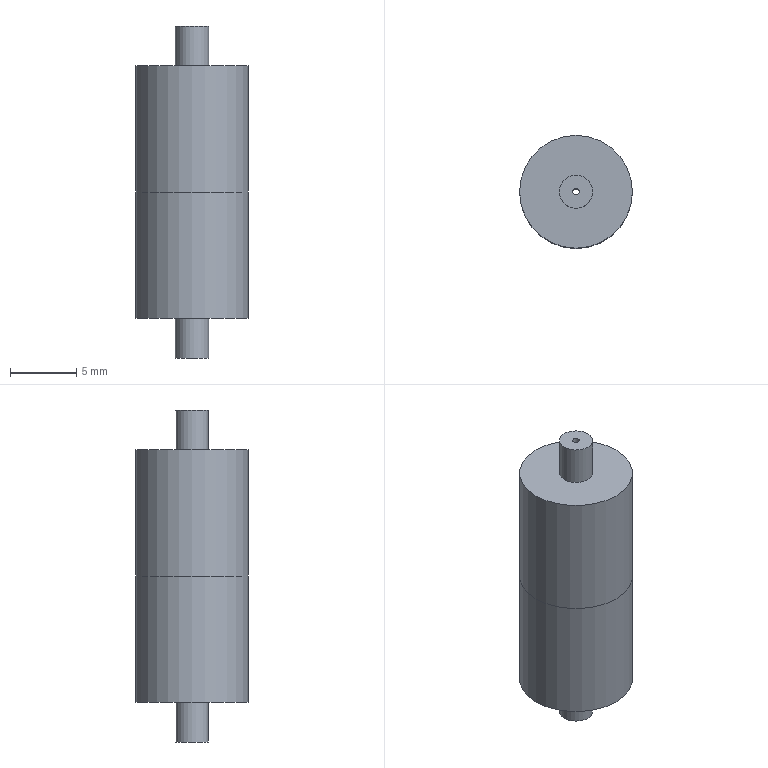Component | NX | MODEL6 | 2 solids | 12 faces | box 8.49 x 8.49 x 25 mm | volume 1101 mm3 | plane 6 | cylinder 6 | commonest cylinder face diameters 8.493 x2 0.493 x2 2.493 x2
STEP:
#1=CARTESIAN_POINT('',(0.,0.,0.));
#2=DIRECTION('',(0.,0.,1.));
#3=DIRECTION('',(1.,0.,0.));
#4=AXIS2_PLACEMENT_3D('',#1,#2,#3);
#5=CARTESIAN_POINT('',(86.254,-6.878,25.));
#6=VERTEX_POINT('',#5);
#7=CARTESIAN_POINT('',(90.5,-6.878,25.));
#8=DIRECTION('',(0.,0.,-1.));
#9=DIRECTION('',(-1.,0.,0.));
#10=AXIS2_PLACEMENT_3D('',#7,#8,#9);
#11=CIRCLE('',#10,4.247);
#12=CARTESIAN_POINT('',(90.5,-5.631,25.));
#13=DIRECTION('',(0.,0.,1.));
#14=DIRECTION('',(-1.,0.,0.));
#15=AXIS2_PLACEMENT_3D('',#12,#13,#14);
#16=PLANE('',#15);
#17=CARTESIAN_POINT('',(4.247,1.247));
#18=CARTESIAN_POINT('',(4.247,-6.109));
#19=CARTESIAN_POINT('',(-2.123,-2.431));
#20=CARTESIAN_POINT('',(-8.493,1.247));
#21=CARTESIAN_POINT('',(-2.123,4.925));
#22=CARTESIAN_POINT('',(4.247,8.602));
#23=CARTESIAN_POINT('',(4.247,1.247));
#24=(BOUNDED_CURVE()B_SPLINE_CURVE(2,(#17,#18,#19,#20,#21,#22,#23),.UNSPECIFIED.,.T.,.F.)B_SPLINE_CURVE_WITH_KNOTS((1,2,2,2,2,1),(-2.094,0.,2.094,4.189,6.283,8.378),.UNSPECIFIED.)CURVE()GEOMETRIC_REPRESENTATION_ITEM()RATIONAL_B_SPLINE_CURVE((1.,0.5,1.,0.5,1.,0.5,1.))REPRESENTATION_ITEM(''));
#25=(GEOMETRIC_REPRESENTATION_CONTEXT(2)PARAMETRIC_REPRESENTATION_CONTEXT()REPRESENTATION_CONTEXT('',''));
#26=DEFINITIONAL_REPRESENTATION('',(#24),#25);
#27=PCURVE('',#16,#26);
#28=CARTESIAN_POINT('',(90.5,-6.878,26.72));
#29=DIRECTION('',(0.,0.,1.));
#30=DIRECTION('',(-1.,0.,0.));
#31=AXIS2_PLACEMENT_3D('',#28,#29,#30);
#32=CYLINDRICAL_SURFACE('',#31,4.247);
#33=CARTESIAN_POINT('',(6.283,-1.72));
#34=DIRECTION('',(-1.,0.));
#35=VECTOR('',#34,1.);
#36=LINE('',#33,#35);
#37=(GEOMETRIC_REPRESENTATION_CONTEXT(2)PARAMETRIC_REPRESENTATION_CONTEXT()REPRESENTATION_CONTEXT('',''));
#38=DEFINITIONAL_REPRESENTATION('',(#36),#37);
#39=PCURVE('',#32,#38);
#40=SURFACE_CURVE('',#11,(#27,#39),.PCURVE_S1.);
#41=EDGE_CURVE('',#6,#6,#40,.T.);
#42=ORIENTED_EDGE('',*,*,#41,.F.);
#43=EDGE_LOOP('',(#42));
#44=FACE_BOUND('',#43,.T.);
#45=CARTESIAN_POINT('',(89.254,-6.878,25.));
#46=VERTEX_POINT('',#45);
#47=CARTESIAN_POINT('',(90.5,-6.878,25.));
#48=DIRECTION('',(0.,0.,-1.));
#49=DIRECTION('',(-1.,0.,0.));
#50=AXIS2_PLACEMENT_3D('',#47,#48,#49);
#51=CIRCLE('',#50,1.247);
#52=CARTESIAN_POINT('',(1.247,1.247));
#53=CARTESIAN_POINT('',(1.247,-0.9127));
#54=CARTESIAN_POINT('',(-0.6234,0.167));
#55=CARTESIAN_POINT('',(-2.493,1.247));
#56=CARTESIAN_POINT('',(-0.6234,2.326));
#57=CARTESIAN_POINT('',(1.247,3.406));
#58=CARTESIAN_POINT('',(1.247,1.247));
#59=(BOUNDED_CURVE()B_SPLINE_CURVE(2,(#52,#53,#54,#55,#56,#57,#58),.UNSPECIFIED.,.T.,.F.)B_SPLINE_CURVE_WITH_KNOTS((1,2,2,2,2,1),(-2.094,0.,2.094,4.189,6.283,8.378),.UNSPECIFIED.)CURVE()GEOMETRIC_REPRESENTATION_ITEM()RATIONAL_B_SPLINE_CURVE((1.,0.5,1.,0.5,1.,0.5,1.))REPRESENTATION_ITEM(''));
#60=(GEOMETRIC_REPRESENTATION_CONTEXT(2)PARAMETRIC_REPRESENTATION_CONTEXT()REPRESENTATION_CONTEXT('',''));
#61=DEFINITIONAL_REPRESENTATION('',(#59),#60);
#62=PCURVE('',#16,#61);
#63=CARTESIAN_POINT('',(90.5,-6.878,26.72));
#64=DIRECTION('',(0.,0.,1.));
#65=DIRECTION('',(-1.,0.,0.));
#66=AXIS2_PLACEMENT_3D('',#63,#64,#65);
#67=CYLINDRICAL_SURFACE('',#66,1.247);
#68=CARTESIAN_POINT('',(6.283,-1.72));
#69=DIRECTION('',(-1.,0.));
#70=VECTOR('',#69,1.);
#71=LINE('',#68,#70);
#72=(GEOMETRIC_REPRESENTATION_CONTEXT(2)PARAMETRIC_REPRESENTATION_CONTEXT()REPRESENTATION_CONTEXT('',''));
#73=DEFINITIONAL_REPRESENTATION('',(#71),#72);
#74=PCURVE('',#67,#73);
#75=SURFACE_CURVE('',#51,(#62,#74),.PCURVE_S1.);
#76=EDGE_CURVE('',#46,#46,#75,.T.);
#77=ORIENTED_EDGE('',*,*,#76,.T.);
#78=EDGE_LOOP('',(#77));
#79=FACE_BOUND('',#78,.T.);
#80=ADVANCED_FACE('',(#44,#79),#16,.T.);
#81=CARTESIAN_POINT('',(86.254,-6.878,15.5));
#82=VERTEX_POINT('',#81);
#83=CARTESIAN_POINT('',(90.5,-6.878,15.5));
#84=DIRECTION('',(0.,0.,-1.));
#85=DIRECTION('',(-1.,0.,0.));
#86=AXIS2_PLACEMENT_3D('',#83,#84,#85);
#87=CIRCLE('',#86,4.247);
#88=CARTESIAN_POINT('',(6.283,-11.22));
#89=DIRECTION('',(-1.,0.));
#90=VECTOR('',#89,1.);
#91=LINE('',#88,#90);
#92=(GEOMETRIC_REPRESENTATION_CONTEXT(2)PARAMETRIC_REPRESENTATION_CONTEXT()REPRESENTATION_CONTEXT('',''));
#93=DEFINITIONAL_REPRESENTATION('',(#91),#92);
#94=PCURVE('',#32,#93);
#95=CARTESIAN_POINT('',(90.5,-2.631,15.5));
#96=DIRECTION('',(0.,0.,-1.));
#97=DIRECTION('',(1.,0.,0.));
#98=AXIS2_PLACEMENT_3D('',#95,#96,#97);
#99=PLANE('',#98);
#100=CARTESIAN_POINT('',(0.,4.247));
#101=DIRECTION('',(-1.,0.));
#102=AXIS2_PLACEMENT_2D('',#100,#101);
#103=CIRCLE('',#102,4.247);
#104=(GEOMETRIC_REPRESENTATION_CONTEXT(2)PARAMETRIC_REPRESENTATION_CONTEXT()REPRESENTATION_CONTEXT('',''));
#105=DEFINITIONAL_REPRESENTATION('',(#103),#104);
#106=PCURVE('',#99,#105);
#107=SURFACE_CURVE('',#87,(#94,#106),.PCURVE_S1.);
#108=EDGE_CURVE('',#82,#82,#107,.T.);
#109=ORIENTED_EDGE('',*,*,#108,.F.);
#110=CARTESIAN_POINT('',(86.254,-6.878,15.5));
#111=CARTESIAN_POINT('',(86.254,-6.878,25.));
#112=B_SPLINE_CURVE_WITH_KNOTS('',1,(#110,#111),.UNSPECIFIED.,.F.,.F.,(2,2),(-11.22,-1.72),.PIECEWISE_BEZIER_KNOTS.);
#113=CARTESIAN_POINT('',(6.283,0.));
#114=DIRECTION('',(0.,1.));
#115=VECTOR('',#114,1.);
#116=LINE('',#113,#115);
#117=(GEOMETRIC_REPRESENTATION_CONTEXT(2)PARAMETRIC_REPRESENTATION_CONTEXT()REPRESENTATION_CONTEXT('',''));
#118=DEFINITIONAL_REPRESENTATION('',(#116),#117);
#119=PCURVE('',#32,#118);
#120=CARTESIAN_POINT('',(0.,0.));
#121=DIRECTION('',(0.,1.));
#122=VECTOR('',#121,1.);
#123=LINE('',#120,#122);
#124=(GEOMETRIC_REPRESENTATION_CONTEXT(2)PARAMETRIC_REPRESENTATION_CONTEXT()REPRESENTATION_CONTEXT('',''));
#125=DEFINITIONAL_REPRESENTATION('',(#123),#124);
#126=PCURVE('',#32,#125);
#127=SEAM_CURVE('',#112,(#119,#126),.PCURVE_S1.);
#128=EDGE_CURVE('',#82,#6,#127,.T.);
#129=ORIENTED_EDGE('',*,*,#128,.T.);
#130=ORIENTED_EDGE('',*,*,#41,.T.);
#131=ORIENTED_EDGE('',*,*,#128,.F.);
#132=EDGE_LOOP('',(#109,#129,#130,#131));
#133=FACE_BOUND('',#132,.T.);
#134=ADVANCED_FACE('',(#133),#32,.T.);
#135=CARTESIAN_POINT('',(90.254,-6.878,15.5));
#136=VERTEX_POINT('',#135);
#137=CARTESIAN_POINT('',(90.5,-6.878,15.5));
#138=DIRECTION('',(0.,0.,-1.));
#139=DIRECTION('',(-1.,0.,0.));
#140=AXIS2_PLACEMENT_3D('',#137,#138,#139);
#141=CIRCLE('',#140,0.2467);
#142=CARTESIAN_POINT('',(0.,4.247));
#143=DIRECTION('',(-1.,0.));
#144=AXIS2_PLACEMENT_2D('',#142,#143);
#145=CIRCLE('',#144,0.2467);
#146=(GEOMETRIC_REPRESENTATION_CONTEXT(2)PARAMETRIC_REPRESENTATION_CONTEXT()REPRESENTATION_CONTEXT('',''));
#147=DEFINITIONAL_REPRESENTATION('',(#145),#146);
#148=PCURVE('',#99,#147);
#149=CARTESIAN_POINT('',(90.5,-6.878,26.72));
#150=DIRECTION('',(0.,0.,1.));
#151=DIRECTION('',(-1.,0.,0.));
#152=AXIS2_PLACEMENT_3D('',#149,#150,#151);
#153=CYLINDRICAL_SURFACE('',#152,0.2467);
#154=CARTESIAN_POINT('',(6.283,-11.22));
#155=DIRECTION('',(-1.,0.));
#156=VECTOR('',#155,1.);
#157=LINE('',#154,#156);
#158=(GEOMETRIC_REPRESENTATION_CONTEXT(2)PARAMETRIC_REPRESENTATION_CONTEXT()REPRESENTATION_CONTEXT('',''));
#159=DEFINITIONAL_REPRESENTATION('',(#157),#158);
#160=PCURVE('',#153,#159);
#161=SURFACE_CURVE('',#141,(#148,#160),.PCURVE_S1.);
#162=EDGE_CURVE('',#136,#136,#161,.T.);
#163=ORIENTED_EDGE('',*,*,#162,.F.);
#164=EDGE_LOOP('',(#163));
#165=FACE_BOUND('',#164,.T.);
#166=ORIENTED_EDGE('',*,*,#108,.T.);
#167=EDGE_LOOP('',(#166));
#168=FACE_BOUND('',#167,.T.);
#169=ADVANCED_FACE('',(#165,#168),#99,.T.);
#170=CARTESIAN_POINT('',(90.254,-6.878,28.));
#171=VERTEX_POINT('',#170);
#172=CARTESIAN_POINT('',(90.5,-6.878,28.));
#173=DIRECTION('',(0.,0.,-1.));
#174=DIRECTION('',(-1.,0.,0.));
#175=AXIS2_PLACEMENT_3D('',#172,#173,#174);
#176=CIRCLE('',#175,0.2467);
#177=CARTESIAN_POINT('',(6.283,1.28));
#178=DIRECTION('',(-1.,0.));
#179=VECTOR('',#178,1.);
#180=LINE('',#177,#179);
#181=(GEOMETRIC_REPRESENTATION_CONTEXT(2)PARAMETRIC_REPRESENTATION_CONTEXT()REPRESENTATION_CONTEXT('',''));
#182=DEFINITIONAL_REPRESENTATION('',(#180),#181);
#183=PCURVE('',#153,#182);
#184=CARTESIAN_POINT('',(90.5,-6.631,28.));
#185=DIRECTION('',(0.,0.,1.));
#186=DIRECTION('',(-1.,0.,0.));
#187=AXIS2_PLACEMENT_3D('',#184,#185,#186);
#188=PLANE('',#187);
#189=CARTESIAN_POINT('',(0.2467,0.2467));
#190=CARTESIAN_POINT('',(0.2467,-0.1806));
#191=CARTESIAN_POINT('',(-0.1234,0.03306));
#192=CARTESIAN_POINT('',(-0.4935,0.2467));
#193=CARTESIAN_POINT('',(-0.1234,0.4604));
#194=CARTESIAN_POINT('',(0.2467,0.6741));
#195=CARTESIAN_POINT('',(0.2467,0.2467));
#196=(BOUNDED_CURVE()B_SPLINE_CURVE(2,(#189,#190,#191,#192,#193,#194,#195),.UNSPECIFIED.,.T.,.F.)B_SPLINE_CURVE_WITH_KNOTS((1,2,2,2,2,1),(-2.094,0.,2.094,4.189,6.283,8.378),.UNSPECIFIED.)CURVE()GEOMETRIC_REPRESENTATION_ITEM()RATIONAL_B_SPLINE_CURVE((1.,0.5,1.,0.5,1.,0.5,1.))REPRESENTATION_ITEM(''));
#197=(GEOMETRIC_REPRESENTATION_CONTEXT(2)PARAMETRIC_REPRESENTATION_CONTEXT()REPRESENTATION_CONTEXT('',''));
#198=DEFINITIONAL_REPRESENTATION('',(#196),#197);
#199=PCURVE('',#188,#198);
#200=SURFACE_CURVE('',#176,(#183,#199),.PCURVE_S1.);
#201=EDGE_CURVE('',#171,#171,#200,.T.);
#202=ORIENTED_EDGE('',*,*,#201,.T.);
#203=CARTESIAN_POINT('',(90.254,-6.878,15.5));
#204=CARTESIAN_POINT('',(90.254,-6.878,28.));
#205=B_SPLINE_CURVE_WITH_KNOTS('',1,(#203,#204),.UNSPECIFIED.,.F.,.F.,(2,2),(-11.22,1.28),.PIECEWISE_BEZIER_KNOTS.);
#206=CARTESIAN_POINT('',(0.,0.));
#207=DIRECTION('',(0.,1.));
#208=VECTOR('',#207,1.);
#209=LINE('',#206,#208);
#210=(GEOMETRIC_REPRESENTATION_CONTEXT(2)PARAMETRIC_REPRESENTATION_CONTEXT()REPRESENTATION_CONTEXT('',''));
#211=DEFINITIONAL_REPRESENTATION('',(#209),#210);
#212=PCURVE('',#153,#211);
#213=CARTESIAN_POINT('',(6.283,0.));
#214=DIRECTION('',(0.,1.));
#215=VECTOR('',#214,1.);
#216=LINE('',#213,#215);
#217=(GEOMETRIC_REPRESENTATION_CONTEXT(2)PARAMETRIC_REPRESENTATION_CONTEXT()REPRESENTATION_CONTEXT('',''));
#218=DEFINITIONAL_REPRESENTATION('',(#216),#217);
#219=PCURVE('',#153,#218);
#220=SEAM_CURVE('',#205,(#212,#219),.PCURVE_S1.);
#221=EDGE_CURVE('',#136,#171,#220,.T.);
#222=ORIENTED_EDGE('',*,*,#221,.F.);
#223=ORIENTED_EDGE('',*,*,#162,.F.);
#224=ORIENTED_EDGE('',*,*,#221,.T.);
#225=EDGE_LOOP('',(#202,#222,#223,#224));
#226=FACE_BOUND('',#225,.F.);
#227=ADVANCED_FACE('',(#226),#153,.F.);
#228=CARTESIAN_POINT('',(89.254,-6.878,28.));
#229=VERTEX_POINT('',#228);
#230=CARTESIAN_POINT('',(90.5,-6.878,28.));
#231=DIRECTION('',(0.,0.,-1.));
#232=DIRECTION('',(-1.,0.,0.));
#233=AXIS2_PLACEMENT_3D('',#230,#231,#232);
#234=CIRCLE('',#233,1.247);
#235=CARTESIAN_POINT('',(1.247,0.2467));
#236=CARTESIAN_POINT('',(1.247,-1.913));
#237=CARTESIAN_POINT('',(-0.6234,-0.833));
#238=CARTESIAN_POINT('',(-2.493,0.2467));
#239=CARTESIAN_POINT('',(-0.6234,1.326));
#240=CARTESIAN_POINT('',(1.247,2.406));
#241=CARTESIAN_POINT('',(1.247,0.2467));
#242=(BOUNDED_CURVE()B_SPLINE_CURVE(2,(#235,#236,#237,#238,#239,#240,#241),.UNSPECIFIED.,.T.,.F.)B_SPLINE_CURVE_WITH_KNOTS((1,2,2,2,2,1),(-2.094,0.,2.094,4.189,6.283,8.378),.UNSPECIFIED.)CURVE()GEOMETRIC_REPRESENTATION_ITEM()RATIONAL_B_SPLINE_CURVE((1.,0.5,1.,0.5,1.,0.5,1.))REPRESENTATION_ITEM(''));
#243=(GEOMETRIC_REPRESENTATION_CONTEXT(2)PARAMETRIC_REPRESENTATION_CONTEXT()REPRESENTATION_CONTEXT('',''));
#244=DEFINITIONAL_REPRESENTATION('',(#242),#243);
#245=PCURVE('',#188,#244);
#246=CARTESIAN_POINT('',(6.283,1.28));
#247=DIRECTION('',(-1.,0.));
#248=VECTOR('',#247,1.);
#249=LINE('',#246,#248);
#250=(GEOMETRIC_REPRESENTATION_CONTEXT(2)PARAMETRIC_REPRESENTATION_CONTEXT()REPRESENTATION_CONTEXT('',''));
#251=DEFINITIONAL_REPRESENTATION('',(#249),#250);
#252=PCURVE('',#67,#251);
#253=SURFACE_CURVE('',#234,(#245,#252),.PCURVE_S1.);
#254=EDGE_CURVE('',#229,#229,#253,.T.);
#255=ORIENTED_EDGE('',*,*,#254,.F.);
#256=EDGE_LOOP('',(#255));
#257=FACE_BOUND('',#256,.T.);
#258=ORIENTED_EDGE('',*,*,#201,.T.);
#259=EDGE_LOOP('',(#258));
#260=FACE_BOUND('',#259,.T.);
#261=ADVANCED_FACE('',(#257,#260),#188,.T.);
#262=ORIENTED_EDGE('',*,*,#76,.F.);
#263=CARTESIAN_POINT('',(89.254,-6.878,25.));
#264=CARTESIAN_POINT('',(89.254,-6.878,28.));
#265=B_SPLINE_CURVE_WITH_KNOTS('',1,(#263,#264),.UNSPECIFIED.,.F.,.F.,(2,2),(-1.72,1.28),.PIECEWISE_BEZIER_KNOTS.);
#266=CARTESIAN_POINT('',(6.283,0.));
#267=DIRECTION('',(0.,1.));
#268=VECTOR('',#267,1.);
#269=LINE('',#266,#268);
#270=(GEOMETRIC_REPRESENTATION_CONTEXT(2)PARAMETRIC_REPRESENTATION_CONTEXT()REPRESENTATION_CONTEXT('',''));
#271=DEFINITIONAL_REPRESENTATION('',(#269),#270);
#272=PCURVE('',#67,#271);
#273=CARTESIAN_POINT('',(0.,0.));
#274=DIRECTION('',(0.,1.));
#275=VECTOR('',#274,1.);
#276=LINE('',#273,#275);
#277=(GEOMETRIC_REPRESENTATION_CONTEXT(2)PARAMETRIC_REPRESENTATION_CONTEXT()REPRESENTATION_CONTEXT('',''));
#278=DEFINITIONAL_REPRESENTATION('',(#276),#277);
#279=PCURVE('',#67,#278);
#280=SEAM_CURVE('',#265,(#272,#279),.PCURVE_S1.);
#281=EDGE_CURVE('',#46,#229,#280,.T.);
#282=ORIENTED_EDGE('',*,*,#281,.T.);
#283=ORIENTED_EDGE('',*,*,#254,.T.);
#284=ORIENTED_EDGE('',*,*,#281,.F.);
#285=EDGE_LOOP('',(#262,#282,#283,#284));
#286=FACE_BOUND('',#285,.T.);
#287=ADVANCED_FACE('',(#286),#67,.T.);
#288=CLOSED_SHELL('',(#80,#134,#169,#227,#261,#287));
#289=MANIFOLD_SOLID_BREP('',#288);
#290=(LENGTH_UNIT()NAMED_UNIT(*)SI_UNIT(.MILLI.,.METRE.));
#291=UNCERTAINTY_MEASURE_WITH_UNIT(LENGTH_MEASURE(0.00001),#290,'','');
#292=(NAMED_UNIT(*)PLANE_ANGLE_UNIT()SI_UNIT($,.RADIAN.));
#293=(NAMED_UNIT(*)SI_UNIT($,.STERADIAN.)SOLID_ANGLE_UNIT());
#294=(GEOMETRIC_REPRESENTATION_CONTEXT(3)GLOBAL_UNCERTAINTY_ASSIGNED_CONTEXT((#291))GLOBAL_UNIT_ASSIGNED_CONTEXT((#290,#292,#293))REPRESENTATION_CONTEXT('',''));
#295=ADVANCED_BREP_SHAPE_REPRESENTATION('',(#4,#289),#294);
#296=CARTESIAN_POINT('',(0.,0.,0.));
#297=DIRECTION('',(0.,0.,1.));
#298=DIRECTION('',(1.,0.,0.));
#299=AXIS2_PLACEMENT_3D('',#296,#297,#298);
#300=CARTESIAN_POINT('',(0.,0.,0.));
#301=DIRECTION('',(0.,0.,1.));
#302=DIRECTION('',(1.,0.,0.));
#303=AXIS2_PLACEMENT_3D('',#300,#301,#302);
#304=(LENGTH_UNIT()NAMED_UNIT(*)SI_UNIT(.MILLI.,.METRE.));
#305=UNCERTAINTY_MEASURE_WITH_UNIT(LENGTH_MEASURE(0.00001),#304,'','');
#306=(NAMED_UNIT(*)PLANE_ANGLE_UNIT()SI_UNIT($,.RADIAN.));
#307=(NAMED_UNIT(*)SI_UNIT($,.STERADIAN.)SOLID_ANGLE_UNIT());
#308=(GEOMETRIC_REPRESENTATION_CONTEXT(3)GLOBAL_UNCERTAINTY_ASSIGNED_CONTEXT((#305))GLOBAL_UNIT_ASSIGNED_CONTEXT((#304,#306,#307))REPRESENTATION_CONTEXT('',''));
#309=SHAPE_REPRESENTATION('',(#4,#299,#303),#308);
#310=ITEM_DEFINED_TRANSFORMATION('','',#4,#299);
#311=(REPRESENTATION_RELATIONSHIP('','',#295,#309)REPRESENTATION_RELATIONSHIP_WITH_TRANSFORMATION(#310)SHAPE_REPRESENTATION_RELATIONSHIP());
#312=CARTESIAN_POINT('',(86.254,-6.878,6.));
#313=VERTEX_POINT('',#312);
#314=CARTESIAN_POINT('',(90.5,-6.878,6.));
#315=DIRECTION('',(0.,0.,-1.));
#316=DIRECTION('',(-1.,0.,0.));
#317=AXIS2_PLACEMENT_3D('',#314,#315,#316);
#318=CIRCLE('',#317,4.247);
#319=CARTESIAN_POINT('',(90.5,-5.631,6.));
#320=DIRECTION('',(0.,0.,-1.));
#321=DIRECTION('',(-1.,0.,0.));
#322=AXIS2_PLACEMENT_3D('',#319,#320,#321);
#323=PLANE('',#322);
#324=CARTESIAN_POINT('',(0.,-1.247));
#325=DIRECTION('',(1.,0.));
#326=AXIS2_PLACEMENT_2D('',#324,#325);
#327=CIRCLE('',#326,4.247);
#328=(GEOMETRIC_REPRESENTATION_CONTEXT(2)PARAMETRIC_REPRESENTATION_CONTEXT()REPRESENTATION_CONTEXT('',''));
#329=DEFINITIONAL_REPRESENTATION('',(#327),#328);
#330=PCURVE('',#323,#329);
#331=CARTESIAN_POINT('',(90.5,-6.878,4.28));
#332=DIRECTION('',(0.,0.,-1.));
#333=DIRECTION('',(-1.,0.,0.));
#334=AXIS2_PLACEMENT_3D('',#331,#332,#333);
#335=CYLINDRICAL_SURFACE('',#334,4.247);
#336=CARTESIAN_POINT('',(0.,-1.72));
#337=DIRECTION('',(1.,0.));
#338=VECTOR('',#337,1.);
#339=LINE('',#336,#338);
#340=(GEOMETRIC_REPRESENTATION_CONTEXT(2)PARAMETRIC_REPRESENTATION_CONTEXT()REPRESENTATION_CONTEXT('',''));
#341=DEFINITIONAL_REPRESENTATION('',(#339),#340);
#342=PCURVE('',#335,#341);
#343=SURFACE_CURVE('',#318,(#330,#342),.PCURVE_S1.);
#344=EDGE_CURVE('',#313,#313,#343,.T.);
#345=ORIENTED_EDGE('',*,*,#344,.T.);
#346=EDGE_LOOP('',(#345));
#347=FACE_BOUND('',#346,.T.);
#348=CARTESIAN_POINT('',(89.254,-6.878,6.));
#349=VERTEX_POINT('',#348);
#350=CARTESIAN_POINT('',(90.5,-6.878,6.));
#351=DIRECTION('',(0.,0.,-1.));
#352=DIRECTION('',(-1.,0.,0.));
#353=AXIS2_PLACEMENT_3D('',#350,#351,#352);
#354=CIRCLE('',#353,1.247);
#355=CARTESIAN_POINT('',(0.,-1.247));
#356=DIRECTION('',(1.,0.));
#357=AXIS2_PLACEMENT_2D('',#355,#356);
#358=CIRCLE('',#357,1.247);
#359=(GEOMETRIC_REPRESENTATION_CONTEXT(2)PARAMETRIC_REPRESENTATION_CONTEXT()REPRESENTATION_CONTEXT('',''));
#360=DEFINITIONAL_REPRESENTATION('',(#358),#359);
#361=PCURVE('',#323,#360);
#362=CARTESIAN_POINT('',(90.5,-6.878,4.28));
#363=DIRECTION('',(0.,0.,-1.));
#364=DIRECTION('',(-1.,0.,0.));
#365=AXIS2_PLACEMENT_3D('',#362,#363,#364);
#366=CYLINDRICAL_SURFACE('',#365,1.247);
#367=CARTESIAN_POINT('',(0.,-1.72));
#368=DIRECTION('',(1.,0.));
#369=VECTOR('',#368,1.);
#370=LINE('',#367,#369);
#371=(GEOMETRIC_REPRESENTATION_CONTEXT(2)PARAMETRIC_REPRESENTATION_CONTEXT()REPRESENTATION_CONTEXT('',''));
#372=DEFINITIONAL_REPRESENTATION('',(#370),#371);
#373=PCURVE('',#366,#372);
#374=SURFACE_CURVE('',#354,(#361,#373),.PCURVE_S1.);
#375=EDGE_CURVE('',#349,#349,#374,.T.);
#376=ORIENTED_EDGE('',*,*,#375,.F.);
#377=EDGE_LOOP('',(#376));
#378=FACE_BOUND('',#377,.T.);
#379=ADVANCED_FACE('',(#347,#378),#323,.T.);
#380=CARTESIAN_POINT('',(86.254,-6.878,15.5));
#381=VERTEX_POINT('',#380);
#382=CARTESIAN_POINT('',(90.5,-6.878,15.5));
#383=DIRECTION('',(0.,0.,-1.));
#384=DIRECTION('',(-1.,0.,0.));
#385=AXIS2_PLACEMENT_3D('',#382,#383,#384);
#386=CIRCLE('',#385,4.247);
#387=CARTESIAN_POINT('',(0.,-11.22));
#388=DIRECTION('',(1.,0.));
#389=VECTOR('',#388,1.);
#390=LINE('',#387,#389);
#391=(GEOMETRIC_REPRESENTATION_CONTEXT(2)PARAMETRIC_REPRESENTATION_CONTEXT()REPRESENTATION_CONTEXT('',''));
#392=DEFINITIONAL_REPRESENTATION('',(#390),#391);
#393=PCURVE('',#335,#392);
#394=CARTESIAN_POINT('',(90.5,-2.631,15.5));
#395=DIRECTION('',(0.,0.,1.));
#396=DIRECTION('',(1.,0.,0.));
#397=AXIS2_PLACEMENT_3D('',#394,#395,#396);
#398=PLANE('',#397);
#399=CARTESIAN_POINT('',(-4.247,-4.247));
#400=CARTESIAN_POINT('',(-4.247,3.109));
#401=CARTESIAN_POINT('',(2.123,-0.569));
#402=CARTESIAN_POINT('',(8.493,-4.247));
#403=CARTESIAN_POINT('',(2.123,-7.925));
#404=CARTESIAN_POINT('',(-4.247,-11.602));
#405=CARTESIAN_POINT('',(-4.247,-4.247));
#406=(BOUNDED_CURVE()B_SPLINE_CURVE(2,(#399,#400,#401,#402,#403,#404,#405),.UNSPECIFIED.,.T.,.F.)B_SPLINE_CURVE_WITH_KNOTS((1,2,2,2,2,1),(-2.094,0.,2.094,4.189,6.283,8.378),.UNSPECIFIED.)CURVE()GEOMETRIC_REPRESENTATION_ITEM()RATIONAL_B_SPLINE_CURVE((1.,0.5,1.,0.5,1.,0.5,1.))REPRESENTATION_ITEM(''));
#407=(GEOMETRIC_REPRESENTATION_CONTEXT(2)PARAMETRIC_REPRESENTATION_CONTEXT()REPRESENTATION_CONTEXT('',''));
#408=DEFINITIONAL_REPRESENTATION('',(#406),#407);
#409=PCURVE('',#398,#408);
#410=SURFACE_CURVE('',#386,(#393,#409),.PCURVE_S1.);
#411=EDGE_CURVE('',#381,#381,#410,.T.);
#412=ORIENTED_EDGE('',*,*,#411,.T.);
#413=CARTESIAN_POINT('',(86.254,-6.878,15.5));
#414=CARTESIAN_POINT('',(86.254,-6.878,6.));
#415=B_SPLINE_CURVE_WITH_KNOTS('',1,(#413,#414),.UNSPECIFIED.,.F.,.F.,(2,2),(-11.22,-1.72),.PIECEWISE_BEZIER_KNOTS.);
#416=CARTESIAN_POINT('',(6.283,0.));
#417=DIRECTION('',(0.,1.));
#418=VECTOR('',#417,1.);
#419=LINE('',#416,#418);
#420=(GEOMETRIC_REPRESENTATION_CONTEXT(2)PARAMETRIC_REPRESENTATION_CONTEXT()REPRESENTATION_CONTEXT('',''));
#421=DEFINITIONAL_REPRESENTATION('',(#419),#420);
#422=PCURVE('',#335,#421);
#423=CARTESIAN_POINT('',(0.,0.));
#424=DIRECTION('',(0.,1.));
#425=VECTOR('',#424,1.);
#426=LINE('',#423,#425);
#427=(GEOMETRIC_REPRESENTATION_CONTEXT(2)PARAMETRIC_REPRESENTATION_CONTEXT()REPRESENTATION_CONTEXT('',''));
#428=DEFINITIONAL_REPRESENTATION('',(#426),#427);
#429=PCURVE('',#335,#428);
#430=SEAM_CURVE('',#415,(#422,#429),.PCURVE_S1.);
#431=EDGE_CURVE('',#381,#313,#430,.T.);
#432=ORIENTED_EDGE('',*,*,#431,.T.);
#433=ORIENTED_EDGE('',*,*,#344,.F.);
#434=ORIENTED_EDGE('',*,*,#431,.F.);
#435=EDGE_LOOP('',(#412,#432,#433,#434));
#436=FACE_BOUND('',#435,.T.);
#437=ADVANCED_FACE('',(#436),#335,.T.);
#438=CARTESIAN_POINT('',(90.254,-6.878,15.5));
#439=VERTEX_POINT('',#438);
#440=CARTESIAN_POINT('',(90.5,-6.878,15.5));
#441=DIRECTION('',(0.,0.,-1.));
#442=DIRECTION('',(-1.,0.,0.));
#443=AXIS2_PLACEMENT_3D('',#440,#441,#442);
#444=CIRCLE('',#443,0.2467);
#445=CARTESIAN_POINT('',(-0.2467,-4.247));
#446=CARTESIAN_POINT('',(-0.2467,-3.819));
#447=CARTESIAN_POINT('',(0.1234,-4.033));
#448=CARTESIAN_POINT('',(0.4935,-4.247));
#449=CARTESIAN_POINT('',(0.1234,-4.46));
#450=CARTESIAN_POINT('',(-0.2467,-4.674));
#451=CARTESIAN_POINT('',(-0.2467,-4.247));
#452=(BOUNDED_CURVE()B_SPLINE_CURVE(2,(#445,#446,#447,#448,#449,#450,#451),.UNSPECIFIED.,.T.,.F.)B_SPLINE_CURVE_WITH_KNOTS((1,2,2,2,2,1),(-2.094,0.,2.094,4.189,6.283,8.378),.UNSPECIFIED.)CURVE()GEOMETRIC_REPRESENTATION_ITEM()RATIONAL_B_SPLINE_CURVE((1.,0.5,1.,0.5,1.,0.5,1.))REPRESENTATION_ITEM(''));
#453=(GEOMETRIC_REPRESENTATION_CONTEXT(2)PARAMETRIC_REPRESENTATION_CONTEXT()REPRESENTATION_CONTEXT('',''));
#454=DEFINITIONAL_REPRESENTATION('',(#452),#453);
#455=PCURVE('',#398,#454);
#456=CARTESIAN_POINT('',(90.5,-6.878,4.28));
#457=DIRECTION('',(0.,0.,-1.));
#458=DIRECTION('',(-1.,0.,0.));
#459=AXIS2_PLACEMENT_3D('',#456,#457,#458);
#460=CYLINDRICAL_SURFACE('',#459,0.2467);
#461=CARTESIAN_POINT('',(0.,-11.22));
#462=DIRECTION('',(1.,0.));
#463=VECTOR('',#462,1.);
#464=LINE('',#461,#463);
#465=(GEOMETRIC_REPRESENTATION_CONTEXT(2)PARAMETRIC_REPRESENTATION_CONTEXT()REPRESENTATION_CONTEXT('',''));
#466=DEFINITIONAL_REPRESENTATION('',(#464),#465);
#467=PCURVE('',#460,#466);
#468=SURFACE_CURVE('',#444,(#455,#467),.PCURVE_S1.);
#469=EDGE_CURVE('',#439,#439,#468,.T.);
#470=ORIENTED_EDGE('',*,*,#469,.T.);
#471=EDGE_LOOP('',(#470));
#472=FACE_BOUND('',#471,.T.);
#473=ORIENTED_EDGE('',*,*,#411,.F.);
#474=EDGE_LOOP('',(#473));
#475=FACE_BOUND('',#474,.T.);
#476=ADVANCED_FACE('',(#472,#475),#398,.T.);
#477=CARTESIAN_POINT('',(90.254,-6.878,3.));
#478=VERTEX_POINT('',#477);
#479=CARTESIAN_POINT('',(90.5,-6.878,3.));
#480=DIRECTION('',(0.,0.,-1.));
#481=DIRECTION('',(-1.,0.,0.));
#482=AXIS2_PLACEMENT_3D('',#479,#480,#481);
#483=CIRCLE('',#482,0.2467);
#484=CARTESIAN_POINT('',(0.,1.28));
#485=DIRECTION('',(1.,0.));
#486=VECTOR('',#485,1.);
#487=LINE('',#484,#486);
#488=(GEOMETRIC_REPRESENTATION_CONTEXT(2)PARAMETRIC_REPRESENTATION_CONTEXT()REPRESENTATION_CONTEXT('',''));
#489=DEFINITIONAL_REPRESENTATION('',(#487),#488);
#490=PCURVE('',#460,#489);
#491=CARTESIAN_POINT('',(90.5,-6.631,3.));
#492=DIRECTION('',(0.,0.,-1.));
#493=DIRECTION('',(-1.,0.,0.));
#494=AXIS2_PLACEMENT_3D('',#491,#492,#493);
#495=PLANE('',#494);
#496=CARTESIAN_POINT('',(0.,-0.2467));
#497=DIRECTION('',(1.,0.));
#498=AXIS2_PLACEMENT_2D('',#496,#497);
#499=CIRCLE('',#498,0.2467);
#500=(GEOMETRIC_REPRESENTATION_CONTEXT(2)PARAMETRIC_REPRESENTATION_CONTEXT()REPRESENTATION_CONTEXT('',''));
#501=DEFINITIONAL_REPRESENTATION('',(#499),#500);
#502=PCURVE('',#495,#501);
#503=SURFACE_CURVE('',#483,(#490,#502),.PCURVE_S1.);
#504=EDGE_CURVE('',#478,#478,#503,.T.);
#505=ORIENTED_EDGE('',*,*,#504,.F.);
#506=CARTESIAN_POINT('',(90.254,-6.878,15.5));
#507=CARTESIAN_POINT('',(90.254,-6.878,3.));
#508=B_SPLINE_CURVE_WITH_KNOTS('',1,(#506,#507),.UNSPECIFIED.,.F.,.F.,(2,2),(-11.22,1.28),.PIECEWISE_BEZIER_KNOTS.);
#509=CARTESIAN_POINT('',(0.,0.));
#510=DIRECTION('',(0.,1.));
#511=VECTOR('',#510,1.);
#512=LINE('',#509,#511);
#513=(GEOMETRIC_REPRESENTATION_CONTEXT(2)PARAMETRIC_REPRESENTATION_CONTEXT()REPRESENTATION_CONTEXT('',''));
#514=DEFINITIONAL_REPRESENTATION('',(#512),#513);
#515=PCURVE('',#460,#514);
#516=CARTESIAN_POINT('',(6.283,0.));
#517=DIRECTION('',(0.,1.));
#518=VECTOR('',#517,1.);
#519=LINE('',#516,#518);
#520=(GEOMETRIC_REPRESENTATION_CONTEXT(2)PARAMETRIC_REPRESENTATION_CONTEXT()REPRESENTATION_CONTEXT('',''));
#521=DEFINITIONAL_REPRESENTATION('',(#519),#520);
#522=PCURVE('',#460,#521);
#523=SEAM_CURVE('',#508,(#515,#522),.PCURVE_S1.);
#524=EDGE_CURVE('',#439,#478,#523,.T.);
#525=ORIENTED_EDGE('',*,*,#524,.F.);
#526=ORIENTED_EDGE('',*,*,#469,.T.);
#527=ORIENTED_EDGE('',*,*,#524,.T.);
#528=EDGE_LOOP('',(#505,#525,#526,#527));
#529=FACE_BOUND('',#528,.F.);
#530=ADVANCED_FACE('',(#529),#460,.F.);
#531=CARTESIAN_POINT('',(89.254,-6.878,3.));
#532=VERTEX_POINT('',#531);
#533=CARTESIAN_POINT('',(90.5,-6.878,3.));
#534=DIRECTION('',(0.,0.,-1.));
#535=DIRECTION('',(-1.,0.,0.));
#536=AXIS2_PLACEMENT_3D('',#533,#534,#535);
#537=CIRCLE('',#536,1.247);
#538=CARTESIAN_POINT('',(0.,-0.2467));
#539=DIRECTION('',(1.,0.));
#540=AXIS2_PLACEMENT_2D('',#538,#539);
#541=CIRCLE('',#540,1.247);
#542=(GEOMETRIC_REPRESENTATION_CONTEXT(2)PARAMETRIC_REPRESENTATION_CONTEXT()REPRESENTATION_CONTEXT('',''));
#543=DEFINITIONAL_REPRESENTATION('',(#541),#542);
#544=PCURVE('',#495,#543);
#545=CARTESIAN_POINT('',(0.,1.28));
#546=DIRECTION('',(1.,0.));
#547=VECTOR('',#546,1.);
#548=LINE('',#545,#547);
#549=(GEOMETRIC_REPRESENTATION_CONTEXT(2)PARAMETRIC_REPRESENTATION_CONTEXT()REPRESENTATION_CONTEXT('',''));
#550=DEFINITIONAL_REPRESENTATION('',(#548),#549);
#551=PCURVE('',#366,#550);
#552=SURFACE_CURVE('',#537,(#544,#551),.PCURVE_S1.);
#553=EDGE_CURVE('',#532,#532,#552,.T.);
#554=ORIENTED_EDGE('',*,*,#553,.T.);
#555=EDGE_LOOP('',(#554));
#556=FACE_BOUND('',#555,.T.);
#557=ORIENTED_EDGE('',*,*,#504,.F.);
#558=EDGE_LOOP('',(#557));
#559=FACE_BOUND('',#558,.T.);
#560=ADVANCED_FACE('',(#556,#559),#495,.T.);
#561=ORIENTED_EDGE('',*,*,#375,.T.);
#562=CARTESIAN_POINT('',(89.254,-6.878,6.));
#563=CARTESIAN_POINT('',(89.254,-6.878,3.));
#564=B_SPLINE_CURVE_WITH_KNOTS('',1,(#562,#563),.UNSPECIFIED.,.F.,.F.,(2,2),(-1.72,1.28),.PIECEWISE_BEZIER_KNOTS.);
#565=CARTESIAN_POINT('',(6.283,0.));
#566=DIRECTION('',(0.,1.));
#567=VECTOR('',#566,1.);
#568=LINE('',#565,#567);
#569=(GEOMETRIC_REPRESENTATION_CONTEXT(2)PARAMETRIC_REPRESENTATION_CONTEXT()REPRESENTATION_CONTEXT('',''));
#570=DEFINITIONAL_REPRESENTATION('',(#568),#569);
#571=PCURVE('',#366,#570);
#572=CARTESIAN_POINT('',(0.,0.));
#573=DIRECTION('',(0.,1.));
#574=VECTOR('',#573,1.);
#575=LINE('',#572,#574);
#576=(GEOMETRIC_REPRESENTATION_CONTEXT(2)PARAMETRIC_REPRESENTATION_CONTEXT()REPRESENTATION_CONTEXT('',''));
#577=DEFINITIONAL_REPRESENTATION('',(#575),#576);
#578=PCURVE('',#366,#577);
#579=SEAM_CURVE('',#564,(#571,#578),.PCURVE_S1.);
#580=EDGE_CURVE('',#349,#532,#579,.T.);
#581=ORIENTED_EDGE('',*,*,#580,.T.);
#582=ORIENTED_EDGE('',*,*,#553,.F.);
#583=ORIENTED_EDGE('',*,*,#580,.F.);
#584=EDGE_LOOP('',(#561,#581,#582,#583));
#585=FACE_BOUND('',#584,.T.);
#586=ADVANCED_FACE('',(#585),#366,.T.);
#587=CLOSED_SHELL('',(#379,#437,#476,#530,#560,#586));
#588=MANIFOLD_SOLID_BREP('',#587);
#589=(LENGTH_UNIT()NAMED_UNIT(*)SI_UNIT(.MILLI.,.METRE.));
#590=UNCERTAINTY_MEASURE_WITH_UNIT(LENGTH_MEASURE(0.00001),#589,'','');
#591=(NAMED_UNIT(*)PLANE_ANGLE_UNIT()SI_UNIT($,.RADIAN.));
#592=(NAMED_UNIT(*)SI_UNIT($,.STERADIAN.)SOLID_ANGLE_UNIT());
#593=(GEOMETRIC_REPRESENTATION_CONTEXT(3)GLOBAL_UNCERTAINTY_ASSIGNED_CONTEXT((#590))GLOBAL_UNIT_ASSIGNED_CONTEXT((#589,#591,#592))REPRESENTATION_CONTEXT('',''));
#594=ADVANCED_BREP_SHAPE_REPRESENTATION('',(#4,#588),#593);
#595=ITEM_DEFINED_TRANSFORMATION('','',#4,#303);
#596=(REPRESENTATION_RELATIONSHIP('','',#594,#309)REPRESENTATION_RELATIONSHIP_WITH_TRANSFORMATION(#595)SHAPE_REPRESENTATION_RELATIONSHIP());